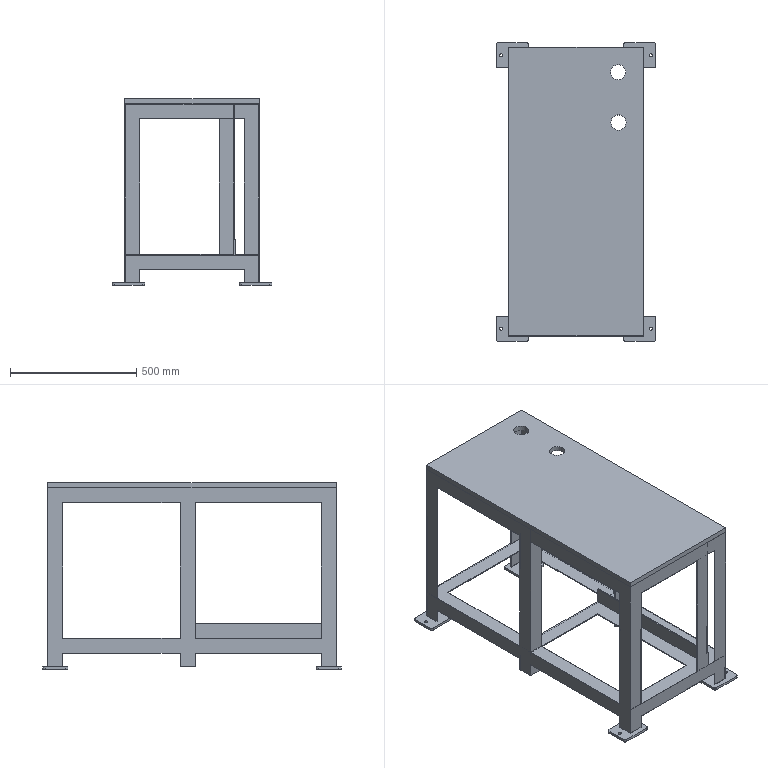Component | NX | SUPPORT_BRACKET | 2 solids | 158 faces | volume 17598772 mm3 | plane 136 | cylinder 22 | commonest cylinder face diameters 20 x16 12.5 x4 60 x2